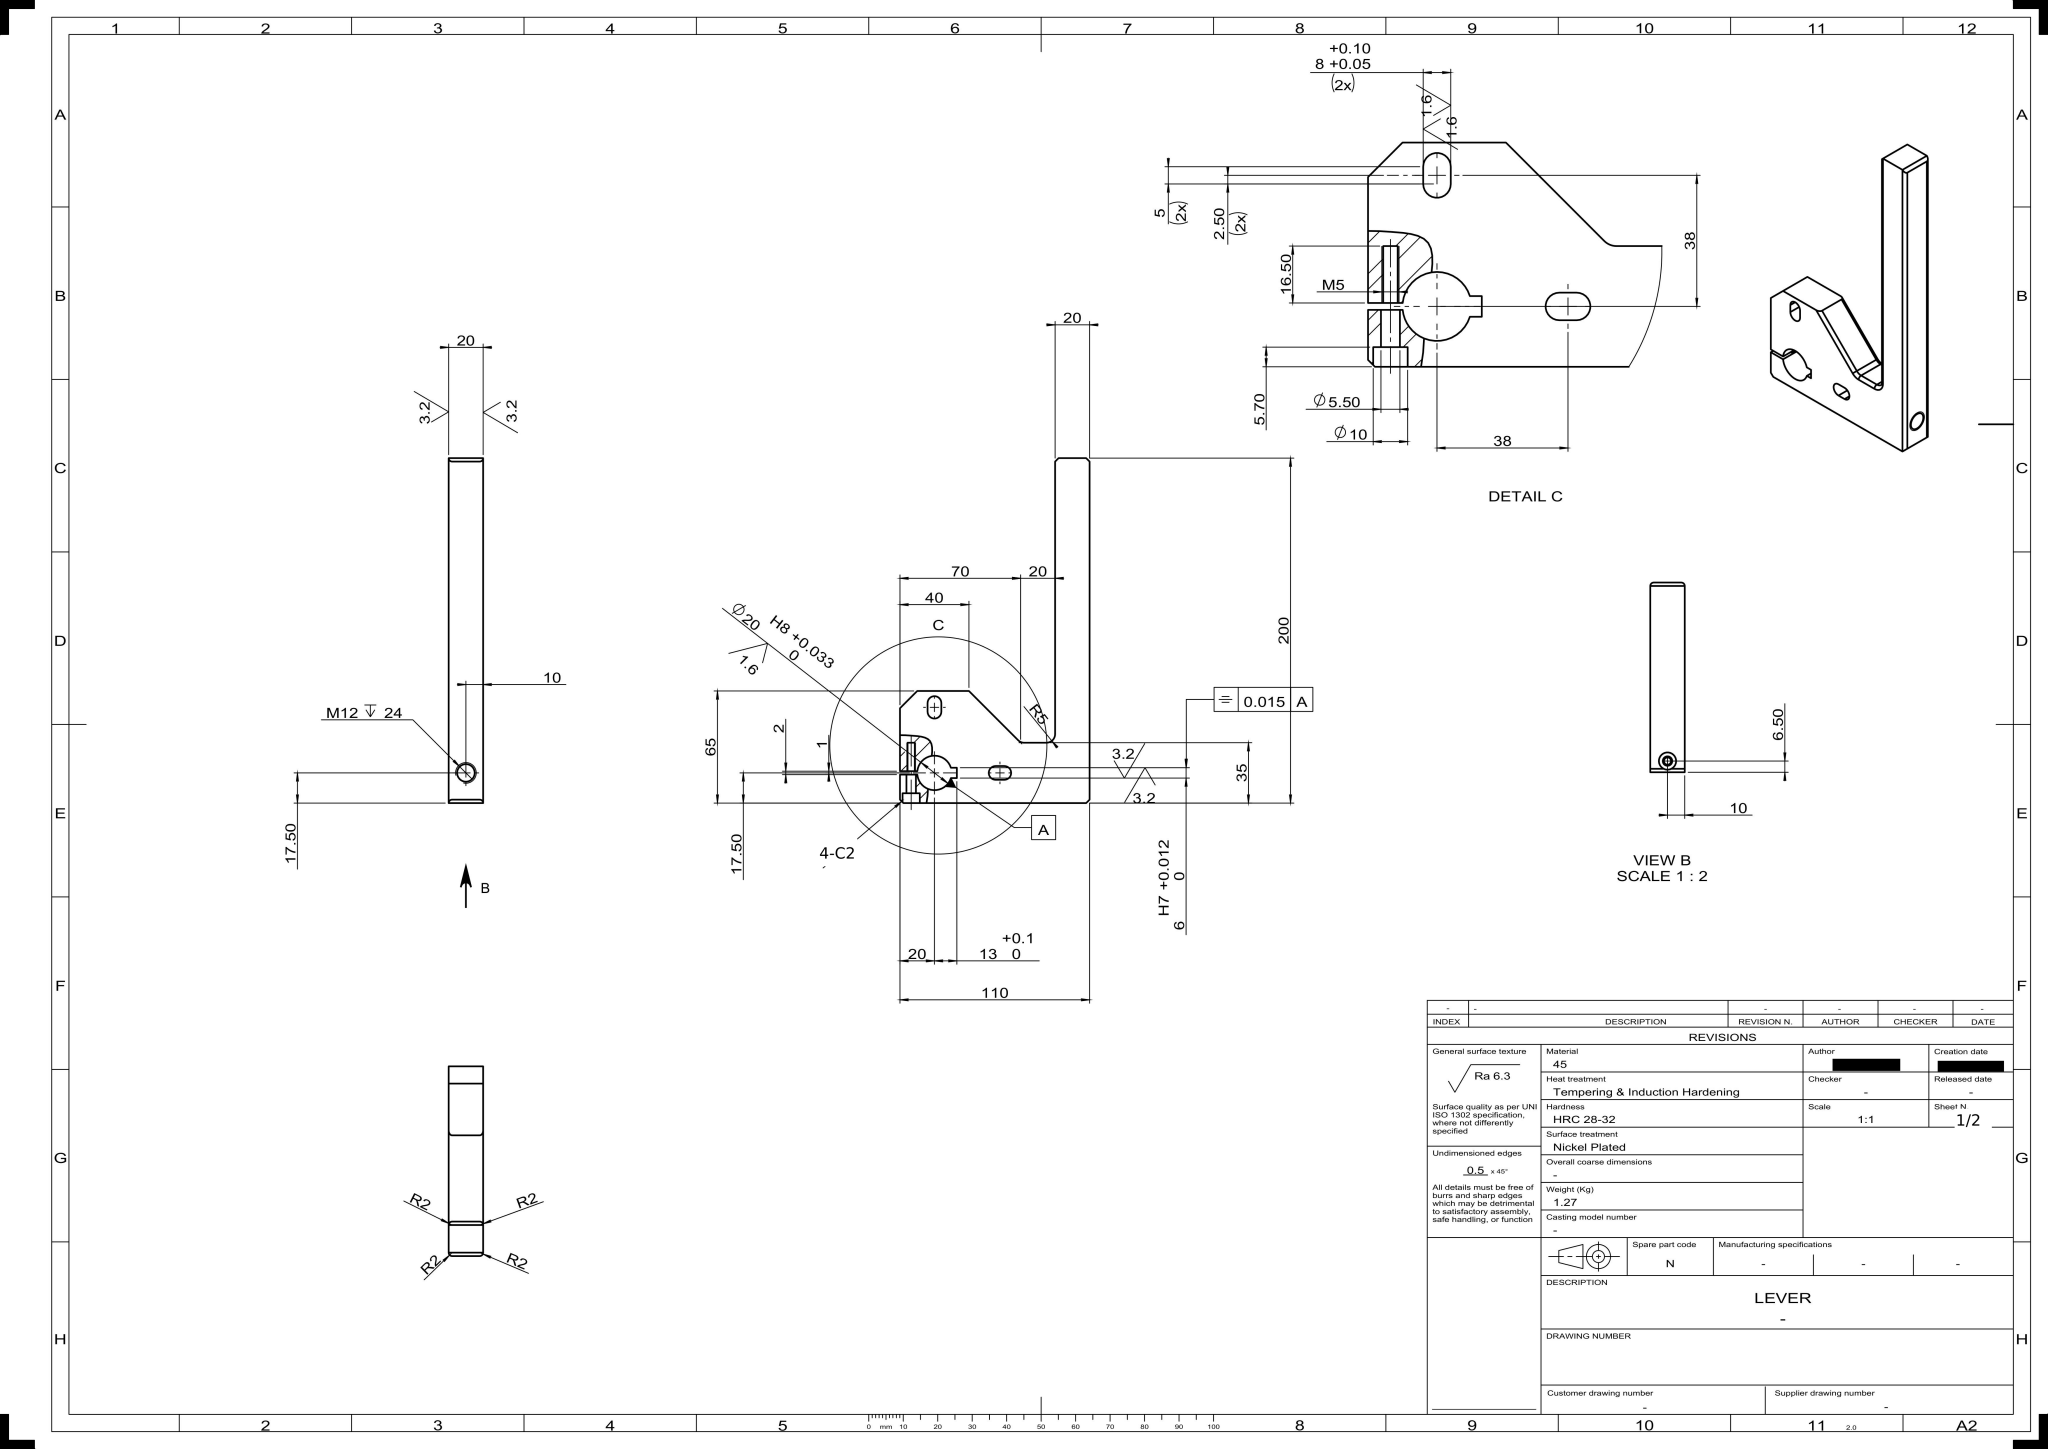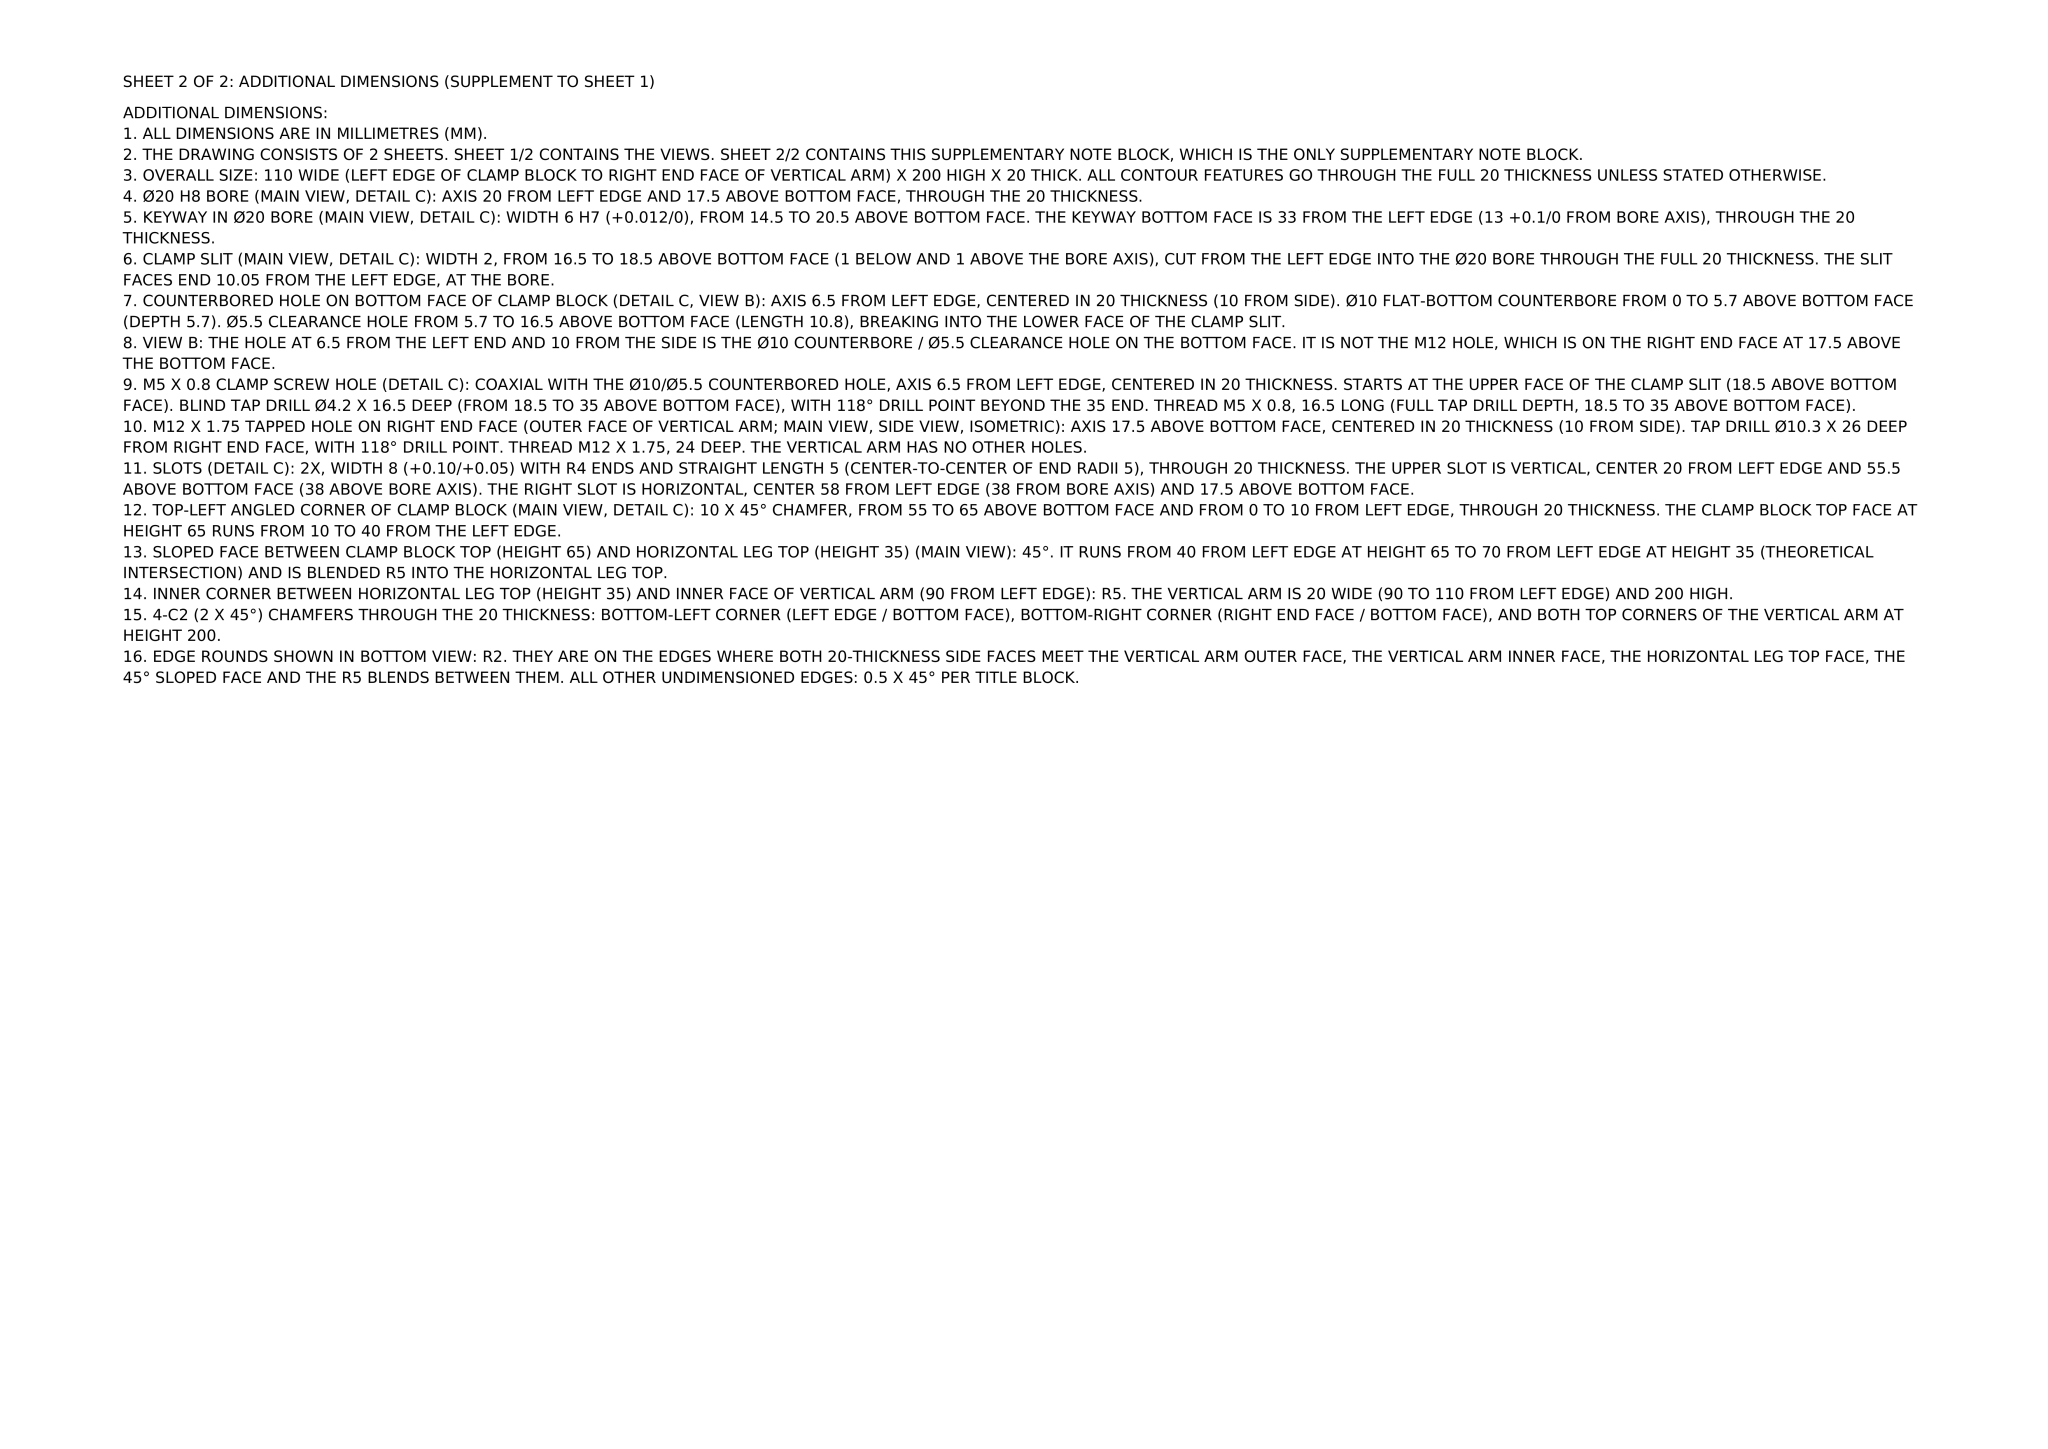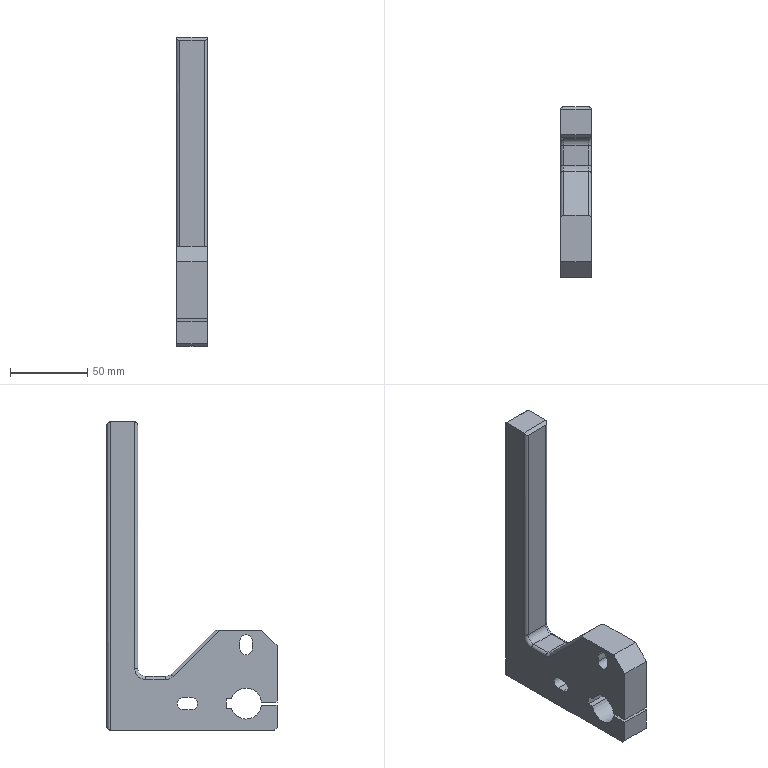Part | NX | mm | 1 solid | 52 faces | box 20 x 110 x 200 mm | volume 160370 mm3 | plane 26 | cylinder 20 | torus 4 | cone 2 | commonest cylinder face diameters 4 x8 8 x4 10 x3 20 x2 5.5 x1 4.2 x1 10.3 x1